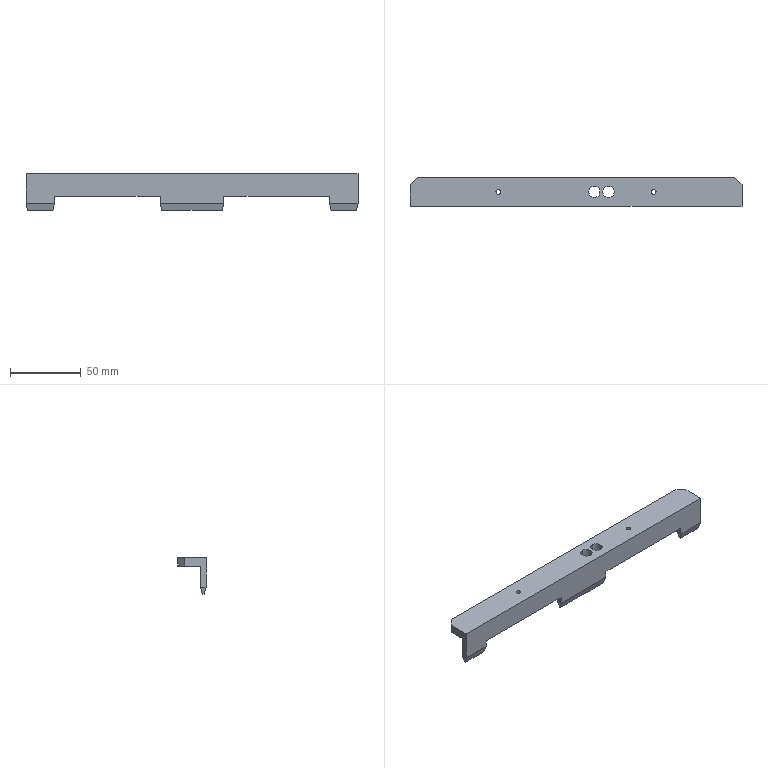Component | SolidWorks | P-SLJ-004-3_P-SLJ-004-004-1 | 1 solid | 38 faces | box 235 x 20 x 26 mm | volume 39477 mm3 | plane 30 | cylinder 8 | commonest cylinder face diameters 8 x4 3.3 x4 | material A3
STEP:
#1=COLOUR_RGB('',0.7922,0.8196,0.9333);
#2=FILL_AREA_STYLE_COLOUR('',#1);
#3=FILL_AREA_STYLE('',(#2));
#4=SURFACE_STYLE_FILL_AREA(#3);
#5=SURFACE_SIDE_STYLE('',(#4));
#6=SURFACE_STYLE_USAGE(.BOTH.,#5);
#7=PRESENTATION_STYLE_ASSIGNMENT((#6));
#8=CARTESIAN_POINT('',(-8.13,-1.614,49.395));
#9=VERTEX_POINT('',#8);
#10=CARTESIAN_POINT('',(-8.13,-1.929,49.395));
#11=VERTEX_POINT('',#10);
#12=CARTESIAN_POINT('',(-8.13,-1.772,49.395));
#13=DIRECTION('',(-0.,-0.,-1.));
#14=DIRECTION('',(0.,-1.,0.));
#15=AXIS2_PLACEMENT_3D('',#12,#13,#14);
#16=CIRCLE('',#15,0.1575);
#17=EDGE_CURVE('',#9,#11,#16,.T.);
#18=ORIENTED_EDGE('',*,*,#17,.F.);
#19=CARTESIAN_POINT('',(-8.13,-1.614,49.159));
#20=VERTEX_POINT('',#19);
#21=CARTESIAN_POINT('',(-8.13,-1.614,49.395));
#22=DIRECTION('',(-0.,-0.,-1.));
#23=VECTOR('',#22,39.37);
#24=LINE('',#21,#23);
#25=EDGE_CURVE('',#9,#20,#24,.T.);
#26=ORIENTED_EDGE('',*,*,#25,.T.);
#27=CARTESIAN_POINT('',(-8.13,-1.929,49.159));
#28=VERTEX_POINT('',#27);
#29=CARTESIAN_POINT('',(-8.13,-1.772,49.159));
#30=DIRECTION('',(-0.,-0.,-1.));
#31=DIRECTION('',(0.,-1.,0.));
#32=AXIS2_PLACEMENT_3D('',#29,#30,#31);
#33=CIRCLE('',#32,0.1575);
#34=EDGE_CURVE('',#20,#28,#33,.T.);
#35=ORIENTED_EDGE('',*,*,#34,.T.);
#36=CARTESIAN_POINT('',(-8.13,-1.929,49.395));
#37=DIRECTION('',(-0.,-0.,-1.));
#38=VECTOR('',#37,39.37);
#39=LINE('',#36,#38);
#40=EDGE_CURVE('',#11,#28,#39,.T.);
#41=ORIENTED_EDGE('',*,*,#40,.F.);
#42=EDGE_LOOP('',(#18,#26,#35,#41));
#43=FACE_OUTER_BOUND('',#42,.T.);
#44=CARTESIAN_POINT('',(-8.13,-1.772,49.395));
#45=DIRECTION('',(-0.,-0.,-1.));
#46=DIRECTION('',(0.,-1.,0.));
#47=AXIS2_PLACEMENT_3D('',#44,#45,#46);
#48=CYLINDRICAL_SURFACE('',#47,0.1575);
#49=ADVANCED_FACE('',(#43),#48,.F.);
#50=CARTESIAN_POINT('',(-7.736,-1.614,49.395));
#51=VERTEX_POINT('',#50);
#52=CARTESIAN_POINT('',(-7.736,-1.929,49.395));
#53=VERTEX_POINT('',#52);
#54=CARTESIAN_POINT('',(-7.736,-1.772,49.395));
#55=DIRECTION('',(-0.,-0.,-1.));
#56=DIRECTION('',(0.,-1.,0.));
#57=AXIS2_PLACEMENT_3D('',#54,#55,#56);
#58=CIRCLE('',#57,0.1575);
#59=EDGE_CURVE('',#51,#53,#58,.T.);
#60=ORIENTED_EDGE('',*,*,#59,.F.);
#61=CARTESIAN_POINT('',(-7.736,-1.614,49.159));
#62=VERTEX_POINT('',#61);
#63=CARTESIAN_POINT('',(-7.736,-1.614,49.395));
#64=DIRECTION('',(-0.,-0.,-1.));
#65=VECTOR('',#64,39.37);
#66=LINE('',#63,#65);
#67=EDGE_CURVE('',#51,#62,#66,.T.);
#68=ORIENTED_EDGE('',*,*,#67,.T.);
#69=CARTESIAN_POINT('',(-7.736,-1.929,49.159));
#70=VERTEX_POINT('',#69);
#71=CARTESIAN_POINT('',(-7.736,-1.772,49.159));
#72=DIRECTION('',(-0.,-0.,-1.));
#73=DIRECTION('',(0.,-1.,0.));
#74=AXIS2_PLACEMENT_3D('',#71,#72,#73);
#75=CIRCLE('',#74,0.1575);
#76=EDGE_CURVE('',#62,#70,#75,.T.);
#77=ORIENTED_EDGE('',*,*,#76,.T.);
#78=CARTESIAN_POINT('',(-7.736,-1.929,49.395));
#79=DIRECTION('',(-0.,-0.,-1.));
#80=VECTOR('',#79,39.37);
#81=LINE('',#78,#80);
#82=EDGE_CURVE('',#53,#70,#81,.T.);
#83=ORIENTED_EDGE('',*,*,#82,.F.);
#84=EDGE_LOOP('',(#60,#68,#77,#83));
#85=FACE_OUTER_BOUND('',#84,.T.);
#86=CARTESIAN_POINT('',(-7.736,-1.772,49.395));
#87=DIRECTION('',(-0.,-0.,-1.));
#88=DIRECTION('',(0.,-1.,0.));
#89=AXIS2_PLACEMENT_3D('',#86,#87,#88);
#90=CYLINDRICAL_SURFACE('',#89,0.1575);
#91=ADVANCED_FACE('',(#85),#90,.F.);
#92=CARTESIAN_POINT('',(-10.872,-1.772,49.159));
#93=VERTEX_POINT('',#92);
#94=CARTESIAN_POINT('',(-10.742,-1.772,49.159));
#95=VERTEX_POINT('',#94);
#96=CARTESIAN_POINT('',(-10.807,-1.772,49.159));
#97=DIRECTION('',(0.,0.,1.));
#98=DIRECTION('',(0.,1.,0.));
#99=AXIS2_PLACEMENT_3D('',#96,#97,#98);
#100=CIRCLE('',#99,0.06496);
#101=EDGE_CURVE('',#93,#95,#100,.T.);
#102=ORIENTED_EDGE('',*,*,#101,.F.);
#103=CARTESIAN_POINT('',(-10.872,-1.772,49.395));
#104=VERTEX_POINT('',#103);
#105=CARTESIAN_POINT('',(-10.872,-1.772,49.395));
#106=DIRECTION('',(0.,-0.,1.));
#107=VECTOR('',#106,39.37);
#108=LINE('',#105,#107);
#109=EDGE_CURVE('',#93,#104,#108,.T.);
#110=ORIENTED_EDGE('',*,*,#109,.T.);
#111=CARTESIAN_POINT('',(-10.742,-1.772,49.395));
#112=VERTEX_POINT('',#111);
#113=CARTESIAN_POINT('',(-10.807,-1.772,49.395));
#114=DIRECTION('',(0.,-0.,1.));
#115=DIRECTION('',(1.,0.,0.));
#116=AXIS2_PLACEMENT_3D('',#113,#114,#115);
#117=CIRCLE('',#116,0.06496);
#118=EDGE_CURVE('',#104,#112,#117,.T.);
#119=ORIENTED_EDGE('',*,*,#118,.T.);
#120=CARTESIAN_POINT('',(-10.742,-1.772,49.395));
#121=DIRECTION('',(0.,-0.,1.));
#122=VECTOR('',#121,39.37);
#123=LINE('',#120,#122);
#124=EDGE_CURVE('',#95,#112,#123,.T.);
#125=ORIENTED_EDGE('',*,*,#124,.F.);
#126=EDGE_LOOP('',(#102,#110,#119,#125));
#127=FACE_OUTER_BOUND('',#126,.T.);
#128=CARTESIAN_POINT('',(-10.807,-1.772,49.395));
#129=DIRECTION('',(0.,-0.,1.));
#130=DIRECTION('',(1.,0.,0.));
#131=AXIS2_PLACEMENT_3D('',#128,#129,#130);
#132=CYLINDRICAL_SURFACE('',#131,0.06496);
#133=ADVANCED_FACE('',(#127),#132,.F.);
#134=CARTESIAN_POINT('',(-6.541,-1.772,49.159));
#135=VERTEX_POINT('',#134);
#136=CARTESIAN_POINT('',(-6.411,-1.772,49.159));
#137=VERTEX_POINT('',#136);
#138=CARTESIAN_POINT('',(-6.476,-1.772,49.159));
#139=DIRECTION('',(0.,0.,1.));
#140=DIRECTION('',(0.,1.,0.));
#141=AXIS2_PLACEMENT_3D('',#138,#139,#140);
#142=CIRCLE('',#141,0.06496);
#143=EDGE_CURVE('',#135,#137,#142,.T.);
#144=ORIENTED_EDGE('',*,*,#143,.F.);
#145=CARTESIAN_POINT('',(-6.541,-1.772,49.395));
#146=VERTEX_POINT('',#145);
#147=CARTESIAN_POINT('',(-6.541,-1.772,49.395));
#148=DIRECTION('',(0.,-0.,1.));
#149=VECTOR('',#148,39.37);
#150=LINE('',#147,#149);
#151=EDGE_CURVE('',#135,#146,#150,.T.);
#152=ORIENTED_EDGE('',*,*,#151,.T.);
#153=CARTESIAN_POINT('',(-6.411,-1.772,49.395));
#154=VERTEX_POINT('',#153);
#155=CARTESIAN_POINT('',(-6.476,-1.772,49.395));
#156=DIRECTION('',(0.,-0.,1.));
#157=DIRECTION('',(1.,0.,0.));
#158=AXIS2_PLACEMENT_3D('',#155,#156,#157);
#159=CIRCLE('',#158,0.06496);
#160=EDGE_CURVE('',#146,#154,#159,.T.);
#161=ORIENTED_EDGE('',*,*,#160,.T.);
#162=CARTESIAN_POINT('',(-6.411,-1.772,49.395));
#163=DIRECTION('',(0.,-0.,1.));
#164=VECTOR('',#163,39.37);
#165=LINE('',#162,#164);
#166=EDGE_CURVE('',#137,#154,#165,.T.);
#167=ORIENTED_EDGE('',*,*,#166,.F.);
#168=EDGE_LOOP('',(#144,#152,#161,#167));
#169=FACE_OUTER_BOUND('',#168,.T.);
#170=CARTESIAN_POINT('',(-6.476,-1.772,49.395));
#171=DIRECTION('',(0.,-0.,1.));
#172=DIRECTION('',(1.,0.,0.));
#173=AXIS2_PLACEMENT_3D('',#170,#171,#172);
#174=CYLINDRICAL_SURFACE('',#173,0.06496);
#175=ADVANCED_FACE('',(#169),#174,.F.);
#176=CARTESIAN_POINT('',(-9.488,-2.067,48.371));
#177=VERTEX_POINT('',#176);
#178=CARTESIAN_POINT('',(-7.795,-2.067,48.371));
#179=VERTEX_POINT('',#178);
#180=CARTESIAN_POINT('',(-13.268,-2.067,48.371));
#181=DIRECTION('',(1.,-0.,-0.));
#182=VECTOR('',#181,39.37);
#183=LINE('',#180,#182);
#184=EDGE_CURVE('',#177,#179,#183,.T.);
#185=ORIENTED_EDGE('',*,*,#184,.F.);
#186=CARTESIAN_POINT('',(-9.528,-2.008,48.568));
#187=VERTEX_POINT('',#186);
#188=CARTESIAN_POINT('',(-9.483,-2.075,48.345));
#189=DIRECTION('',(-0.1881,0.2822,0.9407));
#190=VECTOR('',#189,39.37);
#191=LINE('',#188,#190);
#192=EDGE_CURVE('',#177,#187,#191,.T.);
#193=ORIENTED_EDGE('',*,*,#192,.T.);
#194=CARTESIAN_POINT('',(-7.756,-2.008,48.568));
#195=VERTEX_POINT('',#194);
#196=CARTESIAN_POINT('',(-13.268,-2.008,48.568));
#197=DIRECTION('',(1.,-0.,-0.));
#198=VECTOR('',#197,39.37);
#199=LINE('',#196,#198);
#200=EDGE_CURVE('',#187,#195,#199,.T.);
#201=ORIENTED_EDGE('',*,*,#200,.T.);
#202=CARTESIAN_POINT('',(-7.764,-2.02,48.526));
#203=DIRECTION('',(-0.1881,-0.2822,-0.9407));
#204=VECTOR('',#203,39.37);
#205=LINE('',#202,#204);
#206=EDGE_CURVE('',#195,#179,#205,.T.);
#207=ORIENTED_EDGE('',*,*,#206,.T.);
#208=EDGE_LOOP('',(#185,#193,#201,#207));
#209=FACE_OUTER_BOUND('',#208,.T.);
#210=CARTESIAN_POINT('',(-13.268,-2.067,48.371));
#211=DIRECTION('',(-0.,-0.9578,0.2873));
#212=DIRECTION('',(0.,0.2873,0.9578));
#213=AXIS2_PLACEMENT_3D('',#210,#211,#212);
#214=PLANE('',#213);
#215=ADVANCED_FACE('',(#209),#214,.F.);
#216=CARTESIAN_POINT('',(-7.795,-2.106,48.371));
#217=VERTEX_POINT('',#216);
#218=CARTESIAN_POINT('',(-9.488,-2.106,48.371));
#219=VERTEX_POINT('',#218);
#220=CARTESIAN_POINT('',(-13.268,-2.106,48.371));
#221=DIRECTION('',(-1.,0.,0.));
#222=VECTOR('',#221,39.37);
#223=LINE('',#220,#222);
#224=EDGE_CURVE('',#217,#219,#223,.T.);
#225=ORIENTED_EDGE('',*,*,#224,.T.);
#226=CARTESIAN_POINT('',(-9.488,-2.165,48.371));
#227=DIRECTION('',(0.,1.,0.));
#228=VECTOR('',#227,39.37);
#229=LINE('',#226,#228);
#230=EDGE_CURVE('',#219,#177,#229,.T.);
#231=ORIENTED_EDGE('',*,*,#230,.T.);
#232=ORIENTED_EDGE('',*,*,#184,.T.);
#233=CARTESIAN_POINT('',(-7.795,-2.165,48.371));
#234=DIRECTION('',(-0.,-1.,-0.));
#235=VECTOR('',#234,39.37);
#236=LINE('',#233,#235);
#237=EDGE_CURVE('',#179,#217,#236,.T.);
#238=ORIENTED_EDGE('',*,*,#237,.T.);
#239=EDGE_LOOP('',(#225,#231,#232,#238));
#240=FACE_OUTER_BOUND('',#239,.T.);
#241=CARTESIAN_POINT('',(-13.268,-2.165,48.371));
#242=DIRECTION('',(0.,-0.,1.));
#243=DIRECTION('',(1.,-0.,-0.));
#244=AXIS2_PLACEMENT_3D('',#241,#242,#243);
#245=PLANE('',#244);
#246=ADVANCED_FACE('',(#240),#245,.F.);
#247=CARTESIAN_POINT('',(-4.764,-2.067,48.371));
#248=VERTEX_POINT('',#247);
#249=CARTESIAN_POINT('',(-4.055,-2.067,48.371));
#250=VERTEX_POINT('',#249);
#251=CARTESIAN_POINT('',(-13.268,-2.067,48.371));
#252=DIRECTION('',(1.,-0.,-0.));
#253=VECTOR('',#252,39.37);
#254=LINE('',#251,#253);
#255=EDGE_CURVE('',#248,#250,#254,.T.);
#256=ORIENTED_EDGE('',*,*,#255,.F.);
#257=CARTESIAN_POINT('',(-4.803,-2.008,48.568));
#258=VERTEX_POINT('',#257);
#259=CARTESIAN_POINT('',(-4.759,-2.075,48.345));
#260=DIRECTION('',(-0.1881,0.2822,0.9407));
#261=VECTOR('',#260,39.37);
#262=LINE('',#259,#261);
#263=EDGE_CURVE('',#248,#258,#262,.T.);
#264=ORIENTED_EDGE('',*,*,#263,.T.);
#265=CARTESIAN_POINT('',(-4.016,-2.008,48.568));
#266=VERTEX_POINT('',#265);
#267=CARTESIAN_POINT('',(-13.268,-2.008,48.568));
#268=DIRECTION('',(1.,-0.,-0.));
#269=VECTOR('',#268,39.37);
#270=LINE('',#267,#269);
#271=EDGE_CURVE('',#258,#266,#270,.T.);
#272=ORIENTED_EDGE('',*,*,#271,.T.);
#273=CARTESIAN_POINT('',(-4.06,-2.075,48.345));
#274=DIRECTION('',(-0.1881,-0.2822,-0.9407));
#275=VECTOR('',#274,39.37);
#276=LINE('',#273,#275);
#277=EDGE_CURVE('',#266,#250,#276,.T.);
#278=ORIENTED_EDGE('',*,*,#277,.T.);
#279=EDGE_LOOP('',(#256,#264,#272,#278));
#280=FACE_OUTER_BOUND('',#279,.T.);
#281=CARTESIAN_POINT('',(-13.268,-2.067,48.371));
#282=DIRECTION('',(-0.,-0.9578,0.2873));
#283=DIRECTION('',(0.,0.2873,0.9578));
#284=AXIS2_PLACEMENT_3D('',#281,#282,#283);
#285=PLANE('',#284);
#286=ADVANCED_FACE('',(#280),#285,.F.);
#287=CARTESIAN_POINT('',(-4.055,-2.106,48.371));
#288=VERTEX_POINT('',#287);
#289=CARTESIAN_POINT('',(-4.764,-2.106,48.371));
#290=VERTEX_POINT('',#289);
#291=CARTESIAN_POINT('',(-13.268,-2.106,48.371));
#292=DIRECTION('',(-1.,0.,0.));
#293=VECTOR('',#292,39.37);
#294=LINE('',#291,#293);
#295=EDGE_CURVE('',#288,#290,#294,.T.);
#296=ORIENTED_EDGE('',*,*,#295,.T.);
#297=CARTESIAN_POINT('',(-4.764,-2.165,48.371));
#298=DIRECTION('',(0.,1.,0.));
#299=VECTOR('',#298,39.37);
#300=LINE('',#297,#299);
#301=EDGE_CURVE('',#290,#248,#300,.T.);
#302=ORIENTED_EDGE('',*,*,#301,.T.);
#303=ORIENTED_EDGE('',*,*,#255,.T.);
#304=CARTESIAN_POINT('',(-4.055,-2.165,48.371));
#305=DIRECTION('',(-0.,-1.,-0.));
#306=VECTOR('',#305,39.37);
#307=LINE('',#304,#306);
#308=EDGE_CURVE('',#250,#288,#307,.T.);
#309=ORIENTED_EDGE('',*,*,#308,.T.);
#310=EDGE_LOOP('',(#296,#302,#303,#309));
#311=FACE_OUTER_BOUND('',#310,.T.);
#312=CARTESIAN_POINT('',(-13.268,-2.165,48.371));
#313=DIRECTION('',(0.,-0.,1.));
#314=DIRECTION('',(1.,-0.,-0.));
#315=AXIS2_PLACEMENT_3D('',#312,#313,#314);
#316=PLANE('',#315);
#317=ADVANCED_FACE('',(#311),#316,.F.);
#318=CARTESIAN_POINT('',(-8.13,-1.772,49.395));
#319=DIRECTION('',(-0.,-0.,-1.));
#320=DIRECTION('',(0.,-1.,0.));
#321=AXIS2_PLACEMENT_3D('',#318,#319,#320);
#322=CIRCLE('',#321,0.1575);
#323=EDGE_CURVE('',#11,#9,#322,.T.);
#324=ORIENTED_EDGE('',*,*,#323,.T.);
#325=ORIENTED_EDGE('',*,*,#17,.T.);
#326=EDGE_LOOP('',(#324,#325));
#327=FACE_BOUND('',#326,.T.);
#328=CARTESIAN_POINT('',(-7.736,-1.772,49.395));
#329=DIRECTION('',(-0.,-0.,-1.));
#330=DIRECTION('',(0.,-1.,0.));
#331=AXIS2_PLACEMENT_3D('',#328,#329,#330);
#332=CIRCLE('',#331,0.1575);
#333=EDGE_CURVE('',#53,#51,#332,.T.);
#334=ORIENTED_EDGE('',*,*,#333,.T.);
#335=ORIENTED_EDGE('',*,*,#59,.T.);
#336=EDGE_LOOP('',(#334,#335));
#337=FACE_BOUND('',#336,.T.);
#338=CARTESIAN_POINT('',(-10.807,-1.772,49.395));
#339=DIRECTION('',(0.,-0.,1.));
#340=DIRECTION('',(1.,0.,0.));
#341=AXIS2_PLACEMENT_3D('',#338,#339,#340);
#342=CIRCLE('',#341,0.06496);
#343=EDGE_CURVE('',#112,#104,#342,.T.);
#344=ORIENTED_EDGE('',*,*,#343,.F.);
#345=ORIENTED_EDGE('',*,*,#118,.F.);
#346=EDGE_LOOP('',(#344,#345));
#347=FACE_BOUND('',#346,.T.);
#348=CARTESIAN_POINT('',(-6.476,-1.772,49.395));
#349=DIRECTION('',(0.,-0.,1.));
#350=DIRECTION('',(1.,0.,0.));
#351=AXIS2_PLACEMENT_3D('',#348,#349,#350);
#352=CIRCLE('',#351,0.06496);
#353=EDGE_CURVE('',#154,#146,#352,.T.);
#354=ORIENTED_EDGE('',*,*,#353,.F.);
#355=ORIENTED_EDGE('',*,*,#160,.F.);
#356=EDGE_LOOP('',(#354,#355));
#357=FACE_BOUND('',#356,.T.);
#358=CARTESIAN_POINT('',(-4.016,-2.165,49.395));
#359=VERTEX_POINT('',#358);
#360=CARTESIAN_POINT('',(-4.016,-1.575,49.395));
#361=VERTEX_POINT('',#360);
#362=CARTESIAN_POINT('',(-4.016,-2.165,49.395));
#363=DIRECTION('',(0.,1.,0.));
#364=VECTOR('',#363,39.37);
#365=LINE('',#362,#364);
#366=EDGE_CURVE('',#359,#361,#365,.T.);
#367=ORIENTED_EDGE('',*,*,#366,.T.);
#368=CARTESIAN_POINT('',(-4.213,-1.378,49.395));
#369=VERTEX_POINT('',#368);
#370=CARTESIAN_POINT('',(-4.213,-1.378,49.395));
#371=DIRECTION('',(-0.7071,0.7071,0.));
#372=VECTOR('',#371,39.37);
#373=LINE('',#370,#372);
#374=EDGE_CURVE('',#361,#369,#373,.T.);
#375=ORIENTED_EDGE('',*,*,#374,.T.);
#376=CARTESIAN_POINT('',(-13.071,-1.378,49.395));
#377=VERTEX_POINT('',#376);
#378=CARTESIAN_POINT('',(-13.268,-1.378,49.395));
#379=DIRECTION('',(1.,-0.,-0.));
#380=VECTOR('',#379,39.37);
#381=LINE('',#378,#380);
#382=EDGE_CURVE('',#377,#369,#381,.T.);
#383=ORIENTED_EDGE('',*,*,#382,.F.);
#384=CARTESIAN_POINT('',(-13.268,-1.575,49.395));
#385=VERTEX_POINT('',#384);
#386=CARTESIAN_POINT('',(-13.268,-1.575,49.395));
#387=DIRECTION('',(-0.7071,-0.7071,-0.));
#388=VECTOR('',#387,39.37);
#389=LINE('',#386,#388);
#390=EDGE_CURVE('',#377,#385,#389,.T.);
#391=ORIENTED_EDGE('',*,*,#390,.T.);
#392=CARTESIAN_POINT('',(-13.268,-2.165,49.395));
#393=VERTEX_POINT('',#392);
#394=CARTESIAN_POINT('',(-13.268,-2.165,49.395));
#395=DIRECTION('',(0.,1.,0.));
#396=VECTOR('',#395,39.37);
#397=LINE('',#394,#396);
#398=EDGE_CURVE('',#393,#385,#397,.T.);
#399=ORIENTED_EDGE('',*,*,#398,.F.);
#400=CARTESIAN_POINT('',(-13.268,-2.165,49.395));
#401=DIRECTION('',(1.,-0.,-0.));
#402=VECTOR('',#401,39.37);
#403=LINE('',#400,#402);
#404=EDGE_CURVE('',#393,#359,#403,.T.);
#405=ORIENTED_EDGE('',*,*,#404,.T.);
#406=EDGE_LOOP('',(#367,#375,#383,#391,#399,#405));
#407=FACE_OUTER_BOUND('',#406,.T.);
#408=CARTESIAN_POINT('',(-13.268,-2.165,49.395));
#409=DIRECTION('',(-0.,0.,-1.));
#410=DIRECTION('',(-1.,0.,0.));
#411=AXIS2_PLACEMENT_3D('',#408,#409,#410);
#412=PLANE('',#411);
#413=ADVANCED_FACE('',(#327,#337,#347,#357,#407),#412,.F.);
#414=ORIENTED_EDGE('',*,*,#382,.T.);
#415=CARTESIAN_POINT('',(-4.213,-1.378,49.159));
#416=VERTEX_POINT('',#415);
#417=CARTESIAN_POINT('',(-4.213,-1.378,49.395));
#418=DIRECTION('',(-0.,0.,-1.));
#419=VECTOR('',#418,39.37);
#420=LINE('',#417,#419);
#421=EDGE_CURVE('',#369,#416,#420,.T.);
#422=ORIENTED_EDGE('',*,*,#421,.T.);
#423=CARTESIAN_POINT('',(-13.071,-1.378,49.159));
#424=VERTEX_POINT('',#423);
#425=CARTESIAN_POINT('',(-13.268,-1.378,49.159));
#426=DIRECTION('',(1.,-0.,-0.));
#427=VECTOR('',#426,39.37);
#428=LINE('',#425,#427);
#429=EDGE_CURVE('',#424,#416,#428,.T.);
#430=ORIENTED_EDGE('',*,*,#429,.F.);
#431=CARTESIAN_POINT('',(-13.071,-1.378,49.395));
#432=DIRECTION('',(0.,-0.,1.));
#433=VECTOR('',#432,39.37);
#434=LINE('',#431,#433);
#435=EDGE_CURVE('',#424,#377,#434,.T.);
#436=ORIENTED_EDGE('',*,*,#435,.T.);
#437=EDGE_LOOP('',(#414,#422,#430,#436));
#438=FACE_OUTER_BOUND('',#437,.T.);
#439=CARTESIAN_POINT('',(-13.268,-1.378,49.395));
#440=DIRECTION('',(-0.,-1.,-0.));
#441=DIRECTION('',(1.,-0.,-0.));
#442=AXIS2_PLACEMENT_3D('',#439,#440,#441);
#443=PLANE('',#442);
#444=ADVANCED_FACE('',(#438),#443,.F.);
#445=CARTESIAN_POINT('',(-8.13,-1.772,49.159));
#446=DIRECTION('',(-0.,-0.,-1.));
#447=DIRECTION('',(0.,-1.,0.));
#448=AXIS2_PLACEMENT_3D('',#445,#446,#447);
#449=CIRCLE('',#448,0.1575);
#450=EDGE_CURVE('',#28,#20,#449,.T.);
#451=ORIENTED_EDGE('',*,*,#450,.F.);
#452=ORIENTED_EDGE('',*,*,#34,.F.);
#453=EDGE_LOOP('',(#451,#452));
#454=FACE_BOUND('',#453,.T.);
#455=CARTESIAN_POINT('',(-7.736,-1.772,49.159));
#456=DIRECTION('',(-0.,-0.,-1.));
#457=DIRECTION('',(0.,-1.,0.));
#458=AXIS2_PLACEMENT_3D('',#455,#456,#457);
#459=CIRCLE('',#458,0.1575);
#460=EDGE_CURVE('',#70,#62,#459,.T.);
#461=ORIENTED_EDGE('',*,*,#460,.F.);
#462=ORIENTED_EDGE('',*,*,#76,.F.);
#463=EDGE_LOOP('',(#461,#462));
#464=FACE_BOUND('',#463,.T.);
#465=CARTESIAN_POINT('',(-10.807,-1.772,49.159));
#466=DIRECTION('',(0.,0.,1.));
#467=DIRECTION('',(0.,1.,0.));
#468=AXIS2_PLACEMENT_3D('',#465,#466,#467);
#469=CIRCLE('',#468,0.06496);
#470=EDGE_CURVE('',#95,#93,#469,.T.);
#471=ORIENTED_EDGE('',*,*,#470,.T.);
#472=ORIENTED_EDGE('',*,*,#101,.T.);
#473=EDGE_LOOP('',(#471,#472));
#474=FACE_BOUND('',#473,.T.);
#475=CARTESIAN_POINT('',(-6.476,-1.772,49.159));
#476=DIRECTION('',(0.,0.,1.));
#477=DIRECTION('',(0.,1.,0.));
#478=AXIS2_PLACEMENT_3D('',#475,#476,#477);
#479=CIRCLE('',#478,0.06496);
#480=EDGE_CURVE('',#137,#135,#479,.T.);
#481=ORIENTED_EDGE('',*,*,#480,.T.);
#482=ORIENTED_EDGE('',*,*,#143,.T.);
#483=EDGE_LOOP('',(#481,#482));
#484=FACE_BOUND('',#483,.T.);
#485=ORIENTED_EDGE('',*,*,#429,.T.);
#486=CARTESIAN_POINT('',(-4.016,-1.575,49.159));
#487=VERTEX_POINT('',#486);
#488=CARTESIAN_POINT('',(-4.213,-1.378,49.159));
#489=DIRECTION('',(0.7071,-0.7071,0.));
#490=VECTOR('',#489,39.37);
#491=LINE('',#488,#490);
#492=EDGE_CURVE('',#416,#487,#491,.T.);
#493=ORIENTED_EDGE('',*,*,#492,.T.);
#494=CARTESIAN_POINT('',(-4.016,-2.008,49.159));
#495=VERTEX_POINT('',#494);
#496=CARTESIAN_POINT('',(-4.016,-1.378,49.159));
#497=DIRECTION('',(-0.,-1.,0.));
#498=VECTOR('',#497,39.37);
#499=LINE('',#496,#498);
#500=EDGE_CURVE('',#487,#495,#499,.T.);
#501=ORIENTED_EDGE('',*,*,#500,.T.);
#502=CARTESIAN_POINT('',(-13.268,-2.008,49.159));
#503=VERTEX_POINT('',#502);
#504=CARTESIAN_POINT('',(-13.268,-2.008,49.159));
#505=DIRECTION('',(1.,-0.,-0.));
#506=VECTOR('',#505,39.37);
#507=LINE('',#504,#506);
#508=EDGE_CURVE('',#503,#495,#507,.T.);
#509=ORIENTED_EDGE('',*,*,#508,.F.);
#510=CARTESIAN_POINT('',(-13.268,-1.575,49.159));
#511=VERTEX_POINT('',#510);
#512=CARTESIAN_POINT('',(-13.268,-1.378,49.159));
#513=DIRECTION('',(-0.,-1.,0.));
#514=VECTOR('',#513,39.37);
#515=LINE('',#512,#514);
#516=EDGE_CURVE('',#511,#503,#515,.T.);
#517=ORIENTED_EDGE('',*,*,#516,.F.);
#518=CARTESIAN_POINT('',(-13.268,-1.575,49.159));
#519=DIRECTION('',(0.7071,0.7071,-0.));
#520=VECTOR('',#519,39.37);
#521=LINE('',#518,#520);
#522=EDGE_CURVE('',#511,#424,#521,.T.);
#523=ORIENTED_EDGE('',*,*,#522,.T.);
#524=EDGE_LOOP('',(#485,#493,#501,#509,#517,#523));
#525=FACE_OUTER_BOUND('',#524,.T.);
#526=CARTESIAN_POINT('',(-13.268,-1.378,49.159));
#527=DIRECTION('',(0.,0.,1.));
#528=DIRECTION('',(0.,1.,-0.));
#529=AXIS2_PLACEMENT_3D('',#526,#527,#528);
#530=PLANE('',#529);
#531=ADVANCED_FACE('',(#454,#464,#474,#484,#525),#530,.F.);
#532=ORIENTED_EDGE('',*,*,#200,.F.);
#533=CARTESIAN_POINT('',(-9.528,-2.008,48.765));
#534=VERTEX_POINT('',#533);
#535=CARTESIAN_POINT('',(-9.528,-2.008,48.371));
#536=DIRECTION('',(-0.,0.,-1.));
#537=VECTOR('',#536,39.37);
#538=LINE('',#535,#537);
#539=EDGE_CURVE('',#534,#187,#538,.T.);
#540=ORIENTED_EDGE('',*,*,#539,.F.);
#541=CARTESIAN_POINT('',(-12.48,-2.008,48.765));
#542=VERTEX_POINT('',#541);
#543=CARTESIAN_POINT('',(-9.528,-2.008,48.765));
#544=DIRECTION('',(1.,-0.,-0.));
#545=VECTOR('',#544,39.37);
#546=LINE('',#543,#545);
#547=EDGE_CURVE('',#542,#534,#546,.T.);
#548=ORIENTED_EDGE('',*,*,#547,.F.);
#549=CARTESIAN_POINT('',(-12.48,-2.008,48.568));
#550=VERTEX_POINT('',#549);
#551=CARTESIAN_POINT('',(-12.48,-2.008,48.371));
#552=DIRECTION('',(0.,-0.,1.));
#553=VECTOR('',#552,39.37);
#554=LINE('',#551,#553);
#555=EDGE_CURVE('',#550,#542,#554,.T.);
#556=ORIENTED_EDGE('',*,*,#555,.F.);
#557=CARTESIAN_POINT('',(-13.268,-2.008,48.568));
#558=VERTEX_POINT('',#557);
#559=CARTESIAN_POINT('',(-13.268,-2.008,48.568));
#560=DIRECTION('',(1.,-0.,-0.));
#561=VECTOR('',#560,39.37);
#562=LINE('',#559,#561);
#563=EDGE_CURVE('',#558,#550,#562,.T.);
#564=ORIENTED_EDGE('',*,*,#563,.F.);
#565=CARTESIAN_POINT('',(-13.268,-2.008,48.568));
#566=DIRECTION('',(-0.,0.,-1.));
#567=VECTOR('',#566,39.37);
#568=LINE('',#565,#567);
#569=EDGE_CURVE('',#503,#558,#568,.T.);
#570=ORIENTED_EDGE('',*,*,#569,.F.);
#571=ORIENTED_EDGE('',*,*,#508,.T.);
#572=CARTESIAN_POINT('',(-4.016,-2.008,48.568));
#573=DIRECTION('',(-0.,0.,-1.));
#574=VECTOR('',#573,39.37);
#575=LINE('',#572,#574);
#576=EDGE_CURVE('',#495,#266,#575,.T.);
#577=ORIENTED_EDGE('',*,*,#576,.T.);
#578=ORIENTED_EDGE('',*,*,#271,.F.);
#579=CARTESIAN_POINT('',(-4.803,-2.008,48.765));
#580=VERTEX_POINT('',#579);
#581=CARTESIAN_POINT('',(-4.803,-2.008,48.371));
#582=DIRECTION('',(-0.,0.,-1.));
#583=VECTOR('',#582,39.37);
#584=LINE('',#581,#583);
#585=EDGE_CURVE('',#580,#258,#584,.T.);
#586=ORIENTED_EDGE('',*,*,#585,.F.);
#587=CARTESIAN_POINT('',(-7.756,-2.008,48.765));
#588=VERTEX_POINT('',#587);
#589=CARTESIAN_POINT('',(-4.803,-2.008,48.765));
#590=DIRECTION('',(1.,-0.,-0.));
#591=VECTOR('',#590,39.37);
#592=LINE('',#589,#591);
#593=EDGE_CURVE('',#588,#580,#592,.T.);
#594=ORIENTED_EDGE('',*,*,#593,.F.);
#595=CARTESIAN_POINT('',(-7.756,-2.008,48.371));
#596=DIRECTION('',(-0.,-0.,1.));
#597=VECTOR('',#596,39.37);
#598=LINE('',#595,#597);
#599=EDGE_CURVE('',#195,#588,#598,.T.);
#600=ORIENTED_EDGE('',*,*,#599,.F.);
#601=EDGE_LOOP('',(#532,#540,#548,#556,#564,#570,#571,#577,#578,#586,#594,#600));
#602=FACE_OUTER_BOUND('',#601,.T.);
#603=CARTESIAN_POINT('',(-13.268,-2.008,48.568));
#604=DIRECTION('',(-0.,-1.,-0.));
#605=DIRECTION('',(1.,-0.,-0.));
#606=AXIS2_PLACEMENT_3D('',#603,#604,#605);
#607=PLANE('',#606);
#608=ADVANCED_FACE('',(#602),#607,.F.);
#609=CARTESIAN_POINT('',(-13.228,-2.067,48.371));
#610=VERTEX_POINT('',#609);
#611=CARTESIAN_POINT('',(-12.52,-2.067,48.371));
#612=VERTEX_POINT('',#611);
#613=CARTESIAN_POINT('',(-13.268,-2.067,48.371));
#614=DIRECTION('',(1.,-0.,-0.));
#615=VECTOR('',#614,39.37);
#616=LINE('',#613,#615);
#617=EDGE_CURVE('',#610,#612,#616,.T.);
#618=ORIENTED_EDGE('',*,*,#617,.F.);
#619=CARTESIAN_POINT('',(-13.259,-2.02,48.526));
#620=DIRECTION('',(-0.1881,0.2822,0.9407));
#621=VECTOR('',#620,39.37);
#622=LINE('',#619,#621);
#623=EDGE_CURVE('',#610,#558,#622,.T.);
#624=ORIENTED_EDGE('',*,*,#623,.T.);
#625=ORIENTED_EDGE('',*,*,#563,.T.);
#626=CARTESIAN_POINT('',(-12.489,-2.02,48.526));
#627=DIRECTION('',(-0.1881,-0.2822,-0.9407));
#628=VECTOR('',#627,39.37);
#629=LINE('',#626,#628);
#630=EDGE_CURVE('',#550,#612,#629,.T.);
#631=ORIENTED_EDGE('',*,*,#630,.T.);
#632=EDGE_LOOP('',(#618,#624,#625,#631));
#633=FACE_OUTER_BOUND('',#632,.T.);
#634=CARTESIAN_POINT('',(-13.268,-2.067,48.371));
#635=DIRECTION('',(-0.,-0.9578,0.2873));
#636=DIRECTION('',(0.,0.2873,0.9578));
#637=AXIS2_PLACEMENT_3D('',#634,#635,#636);
#638=PLANE('',#637);
#639=ADVANCED_FACE('',(#633),#638,.F.);
#640=CARTESIAN_POINT('',(-12.52,-2.106,48.371));
#641=VERTEX_POINT('',#640);
#642=CARTESIAN_POINT('',(-13.228,-2.106,48.371));
#643=VERTEX_POINT('',#642);
#644=CARTESIAN_POINT('',(-13.268,-2.106,48.371));
#645=DIRECTION('',(-1.,0.,0.));
#646=VECTOR('',#645,39.37);
#647=LINE('',#644,#646);
#648=EDGE_CURVE('',#641,#643,#647,.T.);
#649=ORIENTED_EDGE('',*,*,#648,.T.);
#650=CARTESIAN_POINT('',(-13.228,-2.067,48.371));
#651=DIRECTION('',(0.,1.,0.));
#652=VECTOR('',#651,39.37);
#653=LINE('',#650,#652);
#654=EDGE_CURVE('',#643,#610,#653,.T.);
#655=ORIENTED_EDGE('',*,*,#654,.T.);
#656=ORIENTED_EDGE('',*,*,#617,.T.);
#657=CARTESIAN_POINT('',(-12.52,-2.165,48.371));
#658=DIRECTION('',(-0.,-1.,-0.));
#659=VECTOR('',#658,39.37);
#660=LINE('',#657,#659);
#661=EDGE_CURVE('',#612,#641,#660,.T.);
#662=ORIENTED_EDGE('',*,*,#661,.T.);
#663=EDGE_LOOP('',(#649,#655,#656,#662));
#664=FACE_OUTER_BOUND('',#663,.T.);
#665=CARTESIAN_POINT('',(-13.268,-2.165,48.371));
#666=DIRECTION('',(0.,-0.,1.));
#667=DIRECTION('',(1.,-0.,-0.));
#668=AXIS2_PLACEMENT_3D('',#665,#666,#667);
#669=PLANE('',#668);
#670=ADVANCED_FACE('',(#664),#669,.F.);
#671=CARTESIAN_POINT('',(-4.803,-2.165,48.765));
#672=VERTEX_POINT('',#671);
#673=CARTESIAN_POINT('',(-4.803,-2.165,48.568));
#674=VERTEX_POINT('',#673);
#675=CARTESIAN_POINT('',(-4.803,-2.165,48.371));
#676=DIRECTION('',(-0.,0.,-1.));
#677=VECTOR('',#676,39.37);
#678=LINE('',#675,#677);
#679=EDGE_CURVE('',#672,#674,#678,.T.);
#680=ORIENTED_EDGE('',*,*,#679,.T.);
#681=CARTESIAN_POINT('',(-4.016,-2.165,48.568));
#682=VERTEX_POINT('',#681);
#683=CARTESIAN_POINT('',(-13.268,-2.165,48.568));
#684=DIRECTION('',(1.,-0.,-0.));
#685=VECTOR('',#684,39.37);
#686=LINE('',#683,#685);
#687=EDGE_CURVE('',#674,#682,#686,.T.);
#688=ORIENTED_EDGE('',*,*,#687,.T.);
#689=CARTESIAN_POINT('',(-4.016,-2.165,49.395));
#690=DIRECTION('',(0.,-0.,1.));
#691=VECTOR('',#690,39.37);
#692=LINE('',#689,#691);
#693=EDGE_CURVE('',#682,#359,#692,.T.);
#694=ORIENTED_EDGE('',*,*,#693,.T.);
#695=ORIENTED_EDGE('',*,*,#404,.F.);
#696=CARTESIAN_POINT('',(-13.268,-2.165,48.568));
#697=VERTEX_POINT('',#696);
#698=CARTESIAN_POINT('',(-13.268,-2.165,49.395));
#699=DIRECTION('',(0.,-0.,1.));
#700=VECTOR('',#699,39.37);
#701=LINE('',#698,#700);
#702=EDGE_CURVE('',#697,#393,#701,.T.);
#703=ORIENTED_EDGE('',*,*,#702,.F.);
#704=CARTESIAN_POINT('',(-12.48,-2.165,48.568));
#705=VERTEX_POINT('',#704);
#706=CARTESIAN_POINT('',(-13.268,-2.165,48.568));
#707=DIRECTION('',(1.,-0.,-0.));
#708=VECTOR('',#707,39.37);
#709=LINE('',#706,#708);
#710=EDGE_CURVE('',#697,#705,#709,.T.);
#711=ORIENTED_EDGE('',*,*,#710,.T.);
#712=CARTESIAN_POINT('',(-12.48,-2.165,48.765));
#713=VERTEX_POINT('',#712);
#714=CARTESIAN_POINT('',(-12.48,-2.165,48.371));
#715=DIRECTION('',(0.,-0.,1.));
#716=VECTOR('',#715,39.37);
#717=LINE('',#714,#716);
#718=EDGE_CURVE('',#705,#713,#717,.T.);
#719=ORIENTED_EDGE('',*,*,#718,.T.);
#720=CARTESIAN_POINT('',(-9.528,-2.165,48.765));
#721=VERTEX_POINT('',#720);
#722=CARTESIAN_POINT('',(-9.528,-2.165,48.765));
#723=DIRECTION('',(1.,-0.,-0.));
#724=VECTOR('',#723,39.37);
#725=LINE('',#722,#724);
#726=EDGE_CURVE('',#713,#721,#725,.T.);
#727=ORIENTED_EDGE('',*,*,#726,.T.);
#728=CARTESIAN_POINT('',(-9.528,-2.165,48.568));
#729=VERTEX_POINT('',#728);
#730=CARTESIAN_POINT('',(-9.528,-2.165,48.371));
#731=DIRECTION('',(-0.,0.,-1.));
#732=VECTOR('',#731,39.37);
#733=LINE('',#730,#732);
#734=EDGE_CURVE('',#721,#729,#733,.T.);
#735=ORIENTED_EDGE('',*,*,#734,.T.);
#736=CARTESIAN_POINT('',(-7.756,-2.165,48.568));
#737=VERTEX_POINT('',#736);
#738=CARTESIAN_POINT('',(-13.268,-2.165,48.568));
#739=DIRECTION('',(1.,-0.,-0.));
#740=VECTOR('',#739,39.37);
#741=LINE('',#738,#740);
#742=EDGE_CURVE('',#729,#737,#741,.T.);
#743=ORIENTED_EDGE('',*,*,#742,.T.);
#744=CARTESIAN_POINT('',(-7.756,-2.165,48.765));
#745=VERTEX_POINT('',#744);
#746=CARTESIAN_POINT('',(-7.756,-2.165,48.371));
#747=DIRECTION('',(-0.,-0.,1.));
#748=VECTOR('',#747,39.37);
#749=LINE('',#746,#748);
#750=EDGE_CURVE('',#737,#745,#749,.T.);
#751=ORIENTED_EDGE('',*,*,#750,.T.);
#752=CARTESIAN_POINT('',(-4.803,-2.165,48.765));
#753=DIRECTION('',(1.,-0.,-0.));
#754=VECTOR('',#753,39.37);
#755=LINE('',#752,#754);
#756=EDGE_CURVE('',#745,#672,#755,.T.);
#757=ORIENTED_EDGE('',*,*,#756,.T.);
#758=EDGE_LOOP('',(#680,#688,#694,#695,#703,#711,#719,#727,#735,#743,#751,#757));
#759=FACE_OUTER_BOUND('',#758,.T.);
#760=CARTESIAN_POINT('',(-13.268,-2.165,49.395));
#761=DIRECTION('',(0.,1.,0.));
#762=DIRECTION('',(-0.,0.,-1.));
#763=AXIS2_PLACEMENT_3D('',#760,#761,#762);
#764=PLANE('',#763);
#765=ADVANCED_FACE('',(#759),#764,.F.);
#766=ORIENTED_EDGE('',*,*,#569,.T.);
#767=CARTESIAN_POINT('',(-13.268,-2.106,48.568));
#768=DIRECTION('',(-0.,-1.,-0.));
#769=VECTOR('',#768,39.37);
#770=LINE('',#767,#769);
#771=EDGE_CURVE('',#558,#697,#770,.T.);
#772=ORIENTED_EDGE('',*,*,#771,.T.);
#773=ORIENTED_EDGE('',*,*,#702,.T.);
#774=ORIENTED_EDGE('',*,*,#398,.T.);
#775=CARTESIAN_POINT('',(-13.268,-1.575,49.159));
#776=DIRECTION('',(-0.,0.,-1.));
#777=VECTOR('',#776,39.37);
#778=LINE('',#775,#777);
#779=EDGE_CURVE('',#385,#511,#778,.T.);
#780=ORIENTED_EDGE('',*,*,#779,.T.);
#781=ORIENTED_EDGE('',*,*,#516,.T.);
#782=EDGE_LOOP('',(#766,#772,#773,#774,#780,#781));
#783=FACE_OUTER_BOUND('',#782,.T.);
#784=CARTESIAN_POINT('',(-13.268,-2.165,49.395));
#785=DIRECTION('',(-1.,0.,0.));
#786=DIRECTION('',(0.,-0.,1.));
#787=AXIS2_PLACEMENT_3D('',#784,#785,#786);
#788=PLANE('',#787);
#789=ADVANCED_FACE('',(#783),#788,.T.);
#790=ORIENTED_EDGE('',*,*,#693,.F.);
#791=CARTESIAN_POINT('',(-4.016,-2.165,48.568));
#792=DIRECTION('',(0.,1.,0.));
#793=VECTOR('',#792,39.37);
#794=LINE('',#791,#793);
#795=EDGE_CURVE('',#682,#266,#794,.T.);
#796=ORIENTED_EDGE('',*,*,#795,.T.);
#797=ORIENTED_EDGE('',*,*,#576,.F.);
#798=ORIENTED_EDGE('',*,*,#500,.F.);
#799=CARTESIAN_POINT('',(-4.016,-1.575,49.395));
#800=DIRECTION('',(0.,-0.,1.));
#801=VECTOR('',#800,39.37);
#802=LINE('',#799,#801);
#803=EDGE_CURVE('',#487,#361,#802,.T.);
#804=ORIENTED_EDGE('',*,*,#803,.T.);
#805=ORIENTED_EDGE('',*,*,#366,.F.);
#806=EDGE_LOOP('',(#790,#796,#797,#798,#804,#805));
#807=FACE_OUTER_BOUND('',#806,.T.);
#808=CARTESIAN_POINT('',(-4.016,-2.165,49.395));
#809=DIRECTION('',(-1.,0.,0.));
#810=DIRECTION('',(0.,-0.,1.));
#811=AXIS2_PLACEMENT_3D('',#808,#809,#810);
#812=PLANE('',#811);
#813=ADVANCED_FACE('',(#807),#812,.F.);
#814=ORIENTED_EDGE('',*,*,#151,.F.);
#815=ORIENTED_EDGE('',*,*,#480,.F.);
#816=ORIENTED_EDGE('',*,*,#166,.T.);
#817=ORIENTED_EDGE('',*,*,#353,.T.);
#818=EDGE_LOOP('',(#814,#815,#816,#817));
#819=FACE_OUTER_BOUND('',#818,.T.);
#820=CARTESIAN_POINT('',(-6.476,-1.772,49.395));
#821=DIRECTION('',(0.,-0.,1.));
#822=DIRECTION('',(1.,0.,0.));
#823=AXIS2_PLACEMENT_3D('',#820,#821,#822);
#824=CYLINDRICAL_SURFACE('',#823,0.06496);
#825=ADVANCED_FACE('',(#819),#824,.F.);
#826=ORIENTED_EDGE('',*,*,#109,.F.);
#827=ORIENTED_EDGE('',*,*,#470,.F.);
#828=ORIENTED_EDGE('',*,*,#124,.T.);
#829=ORIENTED_EDGE('',*,*,#343,.T.);
#830=EDGE_LOOP('',(#826,#827,#828,#829));
#831=FACE_OUTER_BOUND('',#830,.T.);
#832=CARTESIAN_POINT('',(-10.807,-1.772,49.395));
#833=DIRECTION('',(0.,-0.,1.));
#834=DIRECTION('',(1.,0.,0.));
#835=AXIS2_PLACEMENT_3D('',#832,#833,#834);
#836=CYLINDRICAL_SURFACE('',#835,0.06496);
#837=ADVANCED_FACE('',(#831),#836,.F.);
#838=ORIENTED_EDGE('',*,*,#585,.T.);
#839=CARTESIAN_POINT('',(-4.803,-2.165,48.568));
#840=DIRECTION('',(-0.,-1.,-0.));
#841=VECTOR('',#840,39.37);
#842=LINE('',#839,#841);
#843=EDGE_CURVE('',#258,#674,#842,.T.);
#844=ORIENTED_EDGE('',*,*,#843,.T.);
#845=ORIENTED_EDGE('',*,*,#679,.F.);
#846=CARTESIAN_POINT('',(-4.803,-2.165,48.765));
#847=DIRECTION('',(0.,1.,0.));
#848=VECTOR('',#847,39.37);
#849=LINE('',#846,#848);
#850=EDGE_CURVE('',#672,#580,#849,.T.);
#851=ORIENTED_EDGE('',*,*,#850,.T.);
#852=EDGE_LOOP('',(#838,#844,#845,#851));
#853=FACE_OUTER_BOUND('',#852,.T.);
#854=CARTESIAN_POINT('',(-4.803,-2.165,48.371));
#855=DIRECTION('',(1.,-0.,-0.));
#856=DIRECTION('',(-0.,0.,-1.));
#857=AXIS2_PLACEMENT_3D('',#854,#855,#856);
#858=PLANE('',#857);
#859=ADVANCED_FACE('',(#853),#858,.F.);
#860=ORIENTED_EDGE('',*,*,#750,.F.);
#861=CARTESIAN_POINT('',(-7.756,-2.165,48.568));
#862=DIRECTION('',(0.,1.,0.));
#863=VECTOR('',#862,39.37);
#864=LINE('',#861,#863);
#865=EDGE_CURVE('',#737,#195,#864,.T.);
#866=ORIENTED_EDGE('',*,*,#865,.T.);
#867=ORIENTED_EDGE('',*,*,#599,.T.);
#868=CARTESIAN_POINT('',(-7.756,-2.165,48.765));
#869=DIRECTION('',(0.,1.,0.));
#870=VECTOR('',#869,39.37);
#871=LINE('',#868,#870);
#872=EDGE_CURVE('',#745,#588,#871,.T.);
#873=ORIENTED_EDGE('',*,*,#872,.F.);
#874=EDGE_LOOP('',(#860,#866,#867,#873));
#875=FACE_OUTER_BOUND('',#874,.T.);
#876=CARTESIAN_POINT('',(-7.756,-2.165,48.371));
#877=DIRECTION('',(-1.,0.,-0.));
#878=DIRECTION('',(-0.,-0.,1.));
#879=AXIS2_PLACEMENT_3D('',#876,#877,#878);
#880=PLANE('',#879);
#881=ADVANCED_FACE('',(#875),#880,.F.);
#882=ORIENTED_EDGE('',*,*,#593,.T.);
#883=ORIENTED_EDGE('',*,*,#850,.F.);
#884=ORIENTED_EDGE('',*,*,#756,.F.);
#885=ORIENTED_EDGE('',*,*,#872,.T.);
#886=EDGE_LOOP('',(#882,#883,#884,#885));
#887=FACE_OUTER_BOUND('',#886,.T.);
#888=CARTESIAN_POINT('',(-4.803,-2.165,48.765));
#889=DIRECTION('',(0.,-0.,1.));
#890=DIRECTION('',(1.,-0.,-0.));
#891=AXIS2_PLACEMENT_3D('',#888,#889,#890);
#892=PLANE('',#891);
#893=ADVANCED_FACE('',(#887),#892,.F.);
#894=ORIENTED_EDGE('',*,*,#539,.T.);
#895=CARTESIAN_POINT('',(-9.528,-2.165,48.568));
#896=DIRECTION('',(-0.,-1.,-0.));
#897=VECTOR('',#896,39.37);
#898=LINE('',#895,#897);
#899=EDGE_CURVE('',#187,#729,#898,.T.);
#900=ORIENTED_EDGE('',*,*,#899,.T.);
#901=ORIENTED_EDGE('',*,*,#734,.F.);
#902=CARTESIAN_POINT('',(-9.528,-2.165,48.765));
#903=DIRECTION('',(0.,1.,0.));
#904=VECTOR('',#903,39.37);
#905=LINE('',#902,#904);
#906=EDGE_CURVE('',#721,#534,#905,.T.);
#907=ORIENTED_EDGE('',*,*,#906,.T.);
#908=EDGE_LOOP('',(#894,#900,#901,#907));
#909=FACE_OUTER_BOUND('',#908,.T.);
#910=CARTESIAN_POINT('',(-9.528,-2.165,48.371));
#911=DIRECTION('',(1.,-0.,-0.));
#912=DIRECTION('',(-0.,0.,-1.));
#913=AXIS2_PLACEMENT_3D('',#910,#911,#912);
#914=PLANE('',#913);
#915=ADVANCED_FACE('',(#909),#914,.F.);
#916=ORIENTED_EDGE('',*,*,#718,.F.);
#917=CARTESIAN_POINT('',(-12.48,-2.165,48.568));
#918=DIRECTION('',(0.,1.,0.));
#919=VECTOR('',#918,39.37);
#920=LINE('',#917,#919);
#921=EDGE_CURVE('',#705,#550,#920,.T.);
#922=ORIENTED_EDGE('',*,*,#921,.T.);
#923=ORIENTED_EDGE('',*,*,#555,.T.);
#924=CARTESIAN_POINT('',(-12.48,-2.165,48.765));
#925=DIRECTION('',(0.,1.,0.));
#926=VECTOR('',#925,39.37);
#927=LINE('',#924,#926);
#928=EDGE_CURVE('',#713,#542,#927,.T.);
#929=ORIENTED_EDGE('',*,*,#928,.F.);
#930=EDGE_LOOP('',(#916,#922,#923,#929));
#931=FACE_OUTER_BOUND('',#930,.T.);
#932=CARTESIAN_POINT('',(-12.48,-2.165,48.371));
#933=DIRECTION('',(-1.,0.,0.));
#934=DIRECTION('',(0.,-0.,1.));
#935=AXIS2_PLACEMENT_3D('',#932,#933,#934);
#936=PLANE('',#935);
#937=ADVANCED_FACE('',(#931),#936,.F.);
#938=ORIENTED_EDGE('',*,*,#547,.T.);
#939=ORIENTED_EDGE('',*,*,#906,.F.);
#940=ORIENTED_EDGE('',*,*,#726,.F.);
#941=ORIENTED_EDGE('',*,*,#928,.T.);
#942=EDGE_LOOP('',(#938,#939,#940,#941));
#943=FACE_OUTER_BOUND('',#942,.T.);
#944=CARTESIAN_POINT('',(-9.528,-2.165,48.765));
#945=DIRECTION('',(0.,-0.,1.));
#946=DIRECTION('',(1.,-0.,-0.));
#947=AXIS2_PLACEMENT_3D('',#944,#945,#946);
#948=PLANE('',#947);
#949=ADVANCED_FACE('',(#943),#948,.F.);
#950=ORIENTED_EDGE('',*,*,#374,.F.);
#951=ORIENTED_EDGE('',*,*,#803,.F.);
#952=ORIENTED_EDGE('',*,*,#492,.F.);
#953=ORIENTED_EDGE('',*,*,#421,.F.);
#954=EDGE_LOOP('',(#950,#951,#952,#953));
#955=FACE_OUTER_BOUND('',#954,.T.);
#956=CARTESIAN_POINT('',(-4.213,-1.378,49.395));
#957=DIRECTION('',(-0.7071,-0.7071,-0.));
#958=DIRECTION('',(-0.,0.,-1.));
#959=AXIS2_PLACEMENT_3D('',#956,#957,#958);
#960=PLANE('',#959);
#961=ADVANCED_FACE('',(#955),#960,.F.);
#962=ORIENTED_EDGE('',*,*,#390,.F.);
#963=ORIENTED_EDGE('',*,*,#435,.F.);
#964=ORIENTED_EDGE('',*,*,#522,.F.);
#965=ORIENTED_EDGE('',*,*,#779,.F.);
#966=EDGE_LOOP('',(#962,#963,#964,#965));
#967=FACE_OUTER_BOUND('',#966,.T.);
#968=CARTESIAN_POINT('',(-13.268,-1.575,49.395));
#969=DIRECTION('',(-0.7071,0.7071,0.));
#970=DIRECTION('',(0.,-0.,1.));
#971=AXIS2_PLACEMENT_3D('',#968,#969,#970);
#972=PLANE('',#971);
#973=ADVANCED_FACE('',(#967),#972,.T.);
#974=ORIENTED_EDGE('',*,*,#687,.F.);
#975=CARTESIAN_POINT('',(-5.103,-2.615,50.066));
#976=DIRECTION('',(0.1881,0.2822,-0.9407));
#977=VECTOR('',#976,39.37);
#978=LINE('',#975,#977);
#979=EDGE_CURVE('',#674,#290,#978,.T.);
#980=ORIENTED_EDGE('',*,*,#979,.T.);
#981=ORIENTED_EDGE('',*,*,#295,.F.);
#982=CARTESIAN_POINT('',(-4.343,-1.674,46.931));
#983=DIRECTION('',(0.1881,-0.2822,0.9407));
#984=VECTOR('',#983,39.37);
#985=LINE('',#982,#984);
#986=EDGE_CURVE('',#288,#682,#985,.T.);
#987=ORIENTED_EDGE('',*,*,#986,.T.);
#988=EDGE_LOOP('',(#974,#980,#981,#987));
#989=FACE_OUTER_BOUND('',#988,.T.);
#990=CARTESIAN_POINT('',(-13.268,-2.165,48.568));
#991=DIRECTION('',(0.,0.9578,0.2873));
#992=DIRECTION('',(1.,-0.,-0.));
#993=AXIS2_PLACEMENT_3D('',#990,#991,#992);
#994=PLANE('',#993);
#995=ADVANCED_FACE('',(#989),#994,.F.);
#996=ORIENTED_EDGE('',*,*,#742,.F.);
#997=CARTESIAN_POINT('',(-9.66,-2.364,49.23));
#998=DIRECTION('',(0.1881,0.2822,-0.9407));
#999=VECTOR('',#998,39.37);
#1000=LINE('',#997,#999);
#1001=EDGE_CURVE('',#729,#219,#1000,.T.);
#1002=ORIENTED_EDGE('',*,*,#1001,.T.);
#1003=ORIENTED_EDGE('',*,*,#224,.F.);
#1004=CARTESIAN_POINT('',(-7.951,-1.873,47.593));
#1005=DIRECTION('',(0.1881,-0.2822,0.9407));
#1006=VECTOR('',#1005,39.37);
#1007=LINE('',#1004,#1006);
#1008=EDGE_CURVE('',#217,#737,#1007,.T.);
#1009=ORIENTED_EDGE('',*,*,#1008,.T.);
#1010=EDGE_LOOP('',(#996,#1002,#1003,#1009));
#1011=FACE_OUTER_BOUND('',#1010,.T.);
#1012=CARTESIAN_POINT('',(-13.268,-2.165,48.568));
#1013=DIRECTION('',(0.,0.9578,0.2873));
#1014=DIRECTION('',(1.,-0.,-0.));
#1015=AXIS2_PLACEMENT_3D('',#1012,#1013,#1014);
#1016=PLANE('',#1015);
#1017=ADVANCED_FACE('',(#1011),#1016,.F.);
#1018=ORIENTED_EDGE('',*,*,#710,.F.);
#1019=CARTESIAN_POINT('',(-13.268,-2.165,48.568));
#1020=DIRECTION('',(0.1881,0.2822,-0.9407));
#1021=VECTOR('',#1020,39.37);
#1022=LINE('',#1019,#1021);
#1023=EDGE_CURVE('',#697,#643,#1022,.T.);
#1024=ORIENTED_EDGE('',*,*,#1023,.T.);
#1025=ORIENTED_EDGE('',*,*,#648,.F.);
#1026=CARTESIAN_POINT('',(-12.508,-2.124,48.429));
#1027=DIRECTION('',(0.1881,-0.2822,0.9407));
#1028=VECTOR('',#1027,39.37);
#1029=LINE('',#1026,#1028);
#1030=EDGE_CURVE('',#641,#705,#1029,.T.);
#1031=ORIENTED_EDGE('',*,*,#1030,.T.);
#1032=EDGE_LOOP('',(#1018,#1024,#1025,#1031));
#1033=FACE_OUTER_BOUND('',#1032,.T.);
#1034=CARTESIAN_POINT('',(-13.268,-2.165,48.568));
#1035=DIRECTION('',(0.,0.9578,0.2873));
#1036=DIRECTION('',(1.,-0.,-0.));
#1037=AXIS2_PLACEMENT_3D('',#1034,#1035,#1036);
#1038=PLANE('',#1037);
#1039=ADVANCED_FACE('',(#1033),#1038,.F.);
#1040=ORIENTED_EDGE('',*,*,#979,.F.);
#1041=ORIENTED_EDGE('',*,*,#843,.F.);
#1042=ORIENTED_EDGE('',*,*,#263,.F.);
#1043=ORIENTED_EDGE('',*,*,#301,.F.);
#1044=EDGE_LOOP('',(#1040,#1041,#1042,#1043));
#1045=FACE_OUTER_BOUND('',#1044,.T.);
#1046=CARTESIAN_POINT('',(-4.764,-2.165,48.371));
#1047=DIRECTION('',(0.9806,-0.,0.1961));
#1048=DIRECTION('',(0.,1.,0.));
#1049=AXIS2_PLACEMENT_3D('',#1046,#1047,#1048);
#1050=PLANE('',#1049);
#1051=ADVANCED_FACE('',(#1045),#1050,.F.);
#1052=ORIENTED_EDGE('',*,*,#277,.F.);
#1053=ORIENTED_EDGE('',*,*,#795,.F.);
#1054=ORIENTED_EDGE('',*,*,#986,.F.);
#1055=ORIENTED_EDGE('',*,*,#308,.F.);
#1056=EDGE_LOOP('',(#1052,#1053,#1054,#1055));
#1057=FACE_OUTER_BOUND('',#1056,.T.);
#1058=CARTESIAN_POINT('',(-4.055,-2.165,48.371));
#1059=DIRECTION('',(-0.9806,0.,0.1961));
#1060=DIRECTION('',(-0.,-1.,-0.));
#1061=AXIS2_PLACEMENT_3D('',#1058,#1059,#1060);
#1062=PLANE('',#1061);
#1063=ADVANCED_FACE('',(#1057),#1062,.F.);
#1064=ORIENTED_EDGE('',*,*,#623,.F.);
#1065=ORIENTED_EDGE('',*,*,#654,.F.);
#1066=ORIENTED_EDGE('',*,*,#1023,.F.);
#1067=ORIENTED_EDGE('',*,*,#771,.F.);
#1068=EDGE_LOOP('',(#1064,#1065,#1066,#1067));
#1069=FACE_OUTER_BOUND('',#1068,.T.);
#1070=CARTESIAN_POINT('',(-13.268,-2.165,48.568));
#1071=DIRECTION('',(-0.9806,0.,-0.1961));
#1072=DIRECTION('',(0.,1.,0.));
#1073=AXIS2_PLACEMENT_3D('',#1070,#1071,#1072);
#1074=PLANE('',#1073);
#1075=ADVANCED_FACE('',(#1069),#1074,.T.);
#1076=ORIENTED_EDGE('',*,*,#1030,.F.);
#1077=ORIENTED_EDGE('',*,*,#661,.F.);
#1078=ORIENTED_EDGE('',*,*,#630,.F.);
#1079=ORIENTED_EDGE('',*,*,#921,.F.);
#1080=EDGE_LOOP('',(#1076,#1077,#1078,#1079));
#1081=FACE_OUTER_BOUND('',#1080,.T.);
#1082=CARTESIAN_POINT('',(-12.48,-2.165,48.568));
#1083=DIRECTION('',(-0.9806,0.,0.1961));
#1084=DIRECTION('',(0.,1.,0.));
#1085=AXIS2_PLACEMENT_3D('',#1082,#1083,#1084);
#1086=PLANE('',#1085);
#1087=ADVANCED_FACE('',(#1081),#1086,.F.);
#1088=ORIENTED_EDGE('',*,*,#1008,.F.);
#1089=ORIENTED_EDGE('',*,*,#237,.F.);
#1090=ORIENTED_EDGE('',*,*,#206,.F.);
#1091=ORIENTED_EDGE('',*,*,#865,.F.);
#1092=EDGE_LOOP('',(#1088,#1089,#1090,#1091));
#1093=FACE_OUTER_BOUND('',#1092,.T.);
#1094=CARTESIAN_POINT('',(-7.756,-2.165,48.568));
#1095=DIRECTION('',(-0.9806,0.,0.1961));
#1096=DIRECTION('',(0.,1.,0.));
#1097=AXIS2_PLACEMENT_3D('',#1094,#1095,#1096);
#1098=PLANE('',#1097);
#1099=ADVANCED_FACE('',(#1093),#1098,.F.);
#1100=ORIENTED_EDGE('',*,*,#1001,.F.);
#1101=ORIENTED_EDGE('',*,*,#899,.F.);
#1102=ORIENTED_EDGE('',*,*,#192,.F.);
#1103=ORIENTED_EDGE('',*,*,#230,.F.);
#1104=EDGE_LOOP('',(#1100,#1101,#1102,#1103));
#1105=FACE_OUTER_BOUND('',#1104,.T.);
#1106=CARTESIAN_POINT('',(-9.488,-2.165,48.371));
#1107=DIRECTION('',(0.9806,-0.,0.1961));
#1108=DIRECTION('',(0.,1.,0.));
#1109=AXIS2_PLACEMENT_3D('',#1106,#1107,#1108);
#1110=PLANE('',#1109);
#1111=ADVANCED_FACE('',(#1105),#1110,.F.);
#1112=ORIENTED_EDGE('',*,*,#67,.F.);
#1113=ORIENTED_EDGE('',*,*,#333,.F.);
#1114=ORIENTED_EDGE('',*,*,#82,.T.);
#1115=ORIENTED_EDGE('',*,*,#460,.T.);
#1116=EDGE_LOOP('',(#1112,#1113,#1114,#1115));
#1117=FACE_OUTER_BOUND('',#1116,.T.);
#1118=CARTESIAN_POINT('',(-7.736,-1.772,49.395));
#1119=DIRECTION('',(-0.,-0.,-1.));
#1120=DIRECTION('',(0.,-1.,0.));
#1121=AXIS2_PLACEMENT_3D('',#1118,#1119,#1120);
#1122=CYLINDRICAL_SURFACE('',#1121,0.1575);
#1123=ADVANCED_FACE('',(#1117),#1122,.F.);
#1124=ORIENTED_EDGE('',*,*,#25,.F.);
#1125=ORIENTED_EDGE('',*,*,#323,.F.);
#1126=ORIENTED_EDGE('',*,*,#40,.T.);
#1127=ORIENTED_EDGE('',*,*,#450,.T.);
#1128=EDGE_LOOP('',(#1124,#1125,#1126,#1127));
#1129=FACE_OUTER_BOUND('',#1128,.T.);
#1130=CARTESIAN_POINT('',(-8.13,-1.772,49.395));
#1131=DIRECTION('',(-0.,-0.,-1.));
#1132=DIRECTION('',(0.,-1.,0.));
#1133=AXIS2_PLACEMENT_3D('',#1130,#1131,#1132);
#1134=CYLINDRICAL_SURFACE('',#1133,0.1575);
#1135=ADVANCED_FACE('',(#1129),#1134,.F.);
#1136=CLOSED_SHELL('',(#49,#91,#133,#175,#215,#246,#286,#317,#413,#444,#531,#608,#639,#670,#765,#789,#813,#825,#837,#859,#881,#893,#915,#937,#949,#961,#973,#995,#1017,#1039,#1051,#1063,#1075,#1087,#1099,#1111,#1123,#1135));
#1137=MANIFOLD_SOLID_BREP('',#1136);
#1138=STYLED_ITEM('',(#7),#1137);
#1139=(LENGTH_UNIT()NAMED_UNIT(*)SI_UNIT($,.METRE.));
#1140=LENGTH_MEASURE_WITH_UNIT(LENGTH_MEASURE(0.0254),#1139);
#1141=DIMENSIONAL_EXPONENTS(1.,0.,0.,0.,0.,0.,0.);
#1142=(CONVERSION_BASED_UNIT('',#1140)LENGTH_UNIT()NAMED_UNIT(#1141));
#1143=UNCERTAINTY_MEASURE_WITH_UNIT(LENGTH_MEASURE(0.00001),#1142,'','');
#1144=(NAMED_UNIT(*)PLANE_ANGLE_UNIT()SI_UNIT($,.RADIAN.));
#1145=(NAMED_UNIT(*)SI_UNIT($,.STERADIAN.)SOLID_ANGLE_UNIT());
#1146=(GEOMETRIC_REPRESENTATION_CONTEXT(3)GLOBAL_UNCERTAINTY_ASSIGNED_CONTEXT((#1143))GLOBAL_UNIT_ASSIGNED_CONTEXT((#1142,#1144,#1145))REPRESENTATION_CONTEXT('',''));
#1147=MECHANICAL_DESIGN_GEOMETRIC_PRESENTATION_REPRESENTATION('',(#1138),#1146);
#1148=PRESENTATION_LAYER_ASSIGNMENT('','',(#1138));
#1149=CARTESIAN_POINT('',(0.,0.,0.));
#1150=DIRECTION('',(0.,0.,1.));
#1151=DIRECTION('',(1.,0.,0.));
#1152=AXIS2_PLACEMENT_3D('',#1149,#1150,#1151);
#1153=(LENGTH_UNIT()NAMED_UNIT(*)SI_UNIT($,.METRE.));
#1154=LENGTH_MEASURE_WITH_UNIT(LENGTH_MEASURE(0.0254),#1153);
#1155=DIMENSIONAL_EXPONENTS(1.,0.,0.,0.,0.,0.,0.);
#1156=(CONVERSION_BASED_UNIT('',#1154)LENGTH_UNIT()NAMED_UNIT(#1155));
#1157=UNCERTAINTY_MEASURE_WITH_UNIT(LENGTH_MEASURE(0.00001),#1156,'','');
#1158=(NAMED_UNIT(*)PLANE_ANGLE_UNIT()SI_UNIT($,.RADIAN.));
#1159=(NAMED_UNIT(*)SI_UNIT($,.STERADIAN.)SOLID_ANGLE_UNIT());
#1160=(GEOMETRIC_REPRESENTATION_CONTEXT(3)GLOBAL_UNCERTAINTY_ASSIGNED_CONTEXT((#1157))GLOBAL_UNIT_ASSIGNED_CONTEXT((#1156,#1158,#1159))REPRESENTATION_CONTEXT('',''));
#1161=ADVANCED_BREP_SHAPE_REPRESENTATION('',(#1137,#1152),#1160);